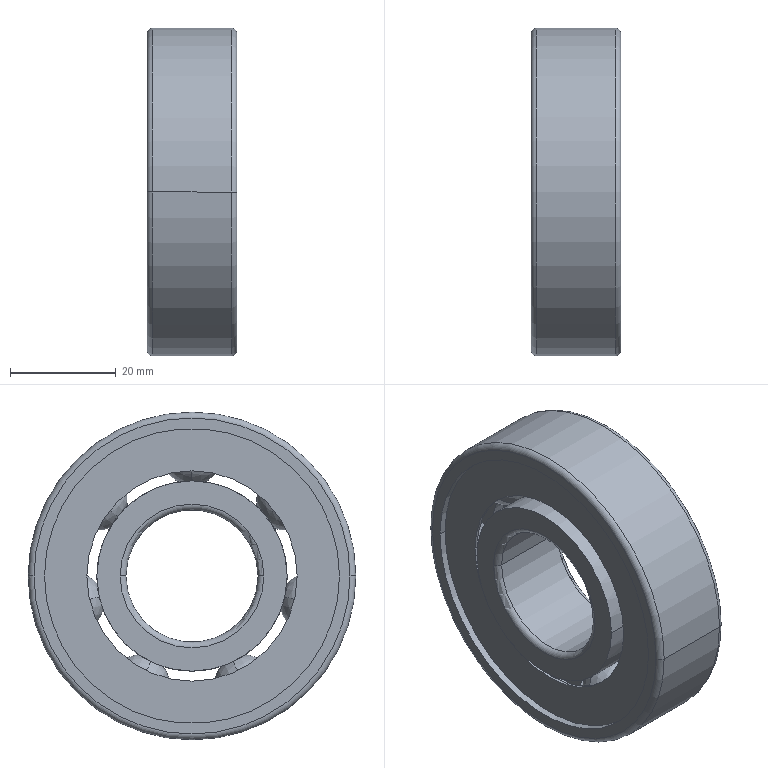Component | SolidWorks | GuideWheelAssembly-2_GB_T276-94DeepGrooveBallBearing6305-2Z-1 | 1 solid | 134 faces | volume 25473 mm3 | sphere 56 | torus 32 | cylinder 24 | plane 22 | commonest cylinder face diameters 55.8 x8 39.795 x4 36 x4 25 x2 62 x2 49.063 x2 42.738 x2